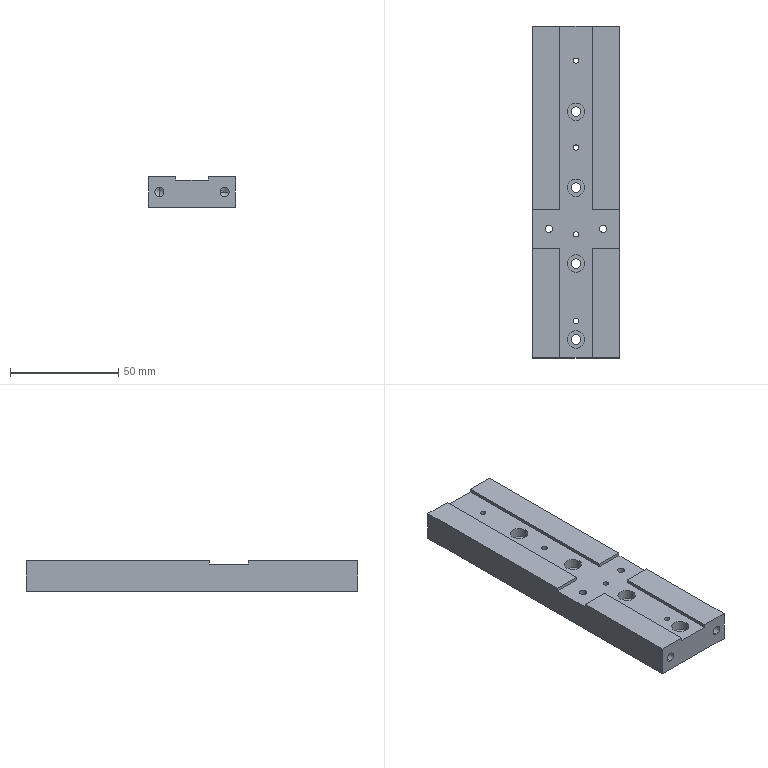Component | SolidWorks | AdhesiveAssemblyFixedPlate-1 | 1 solid | 66 faces | volume 78965 mm3 | cylinder 36 | plane 22 | cone 8 | commonest cylinder face diameters 4.5 x8 2.5 x8 4.2 x8 8 x8 3.3 x4